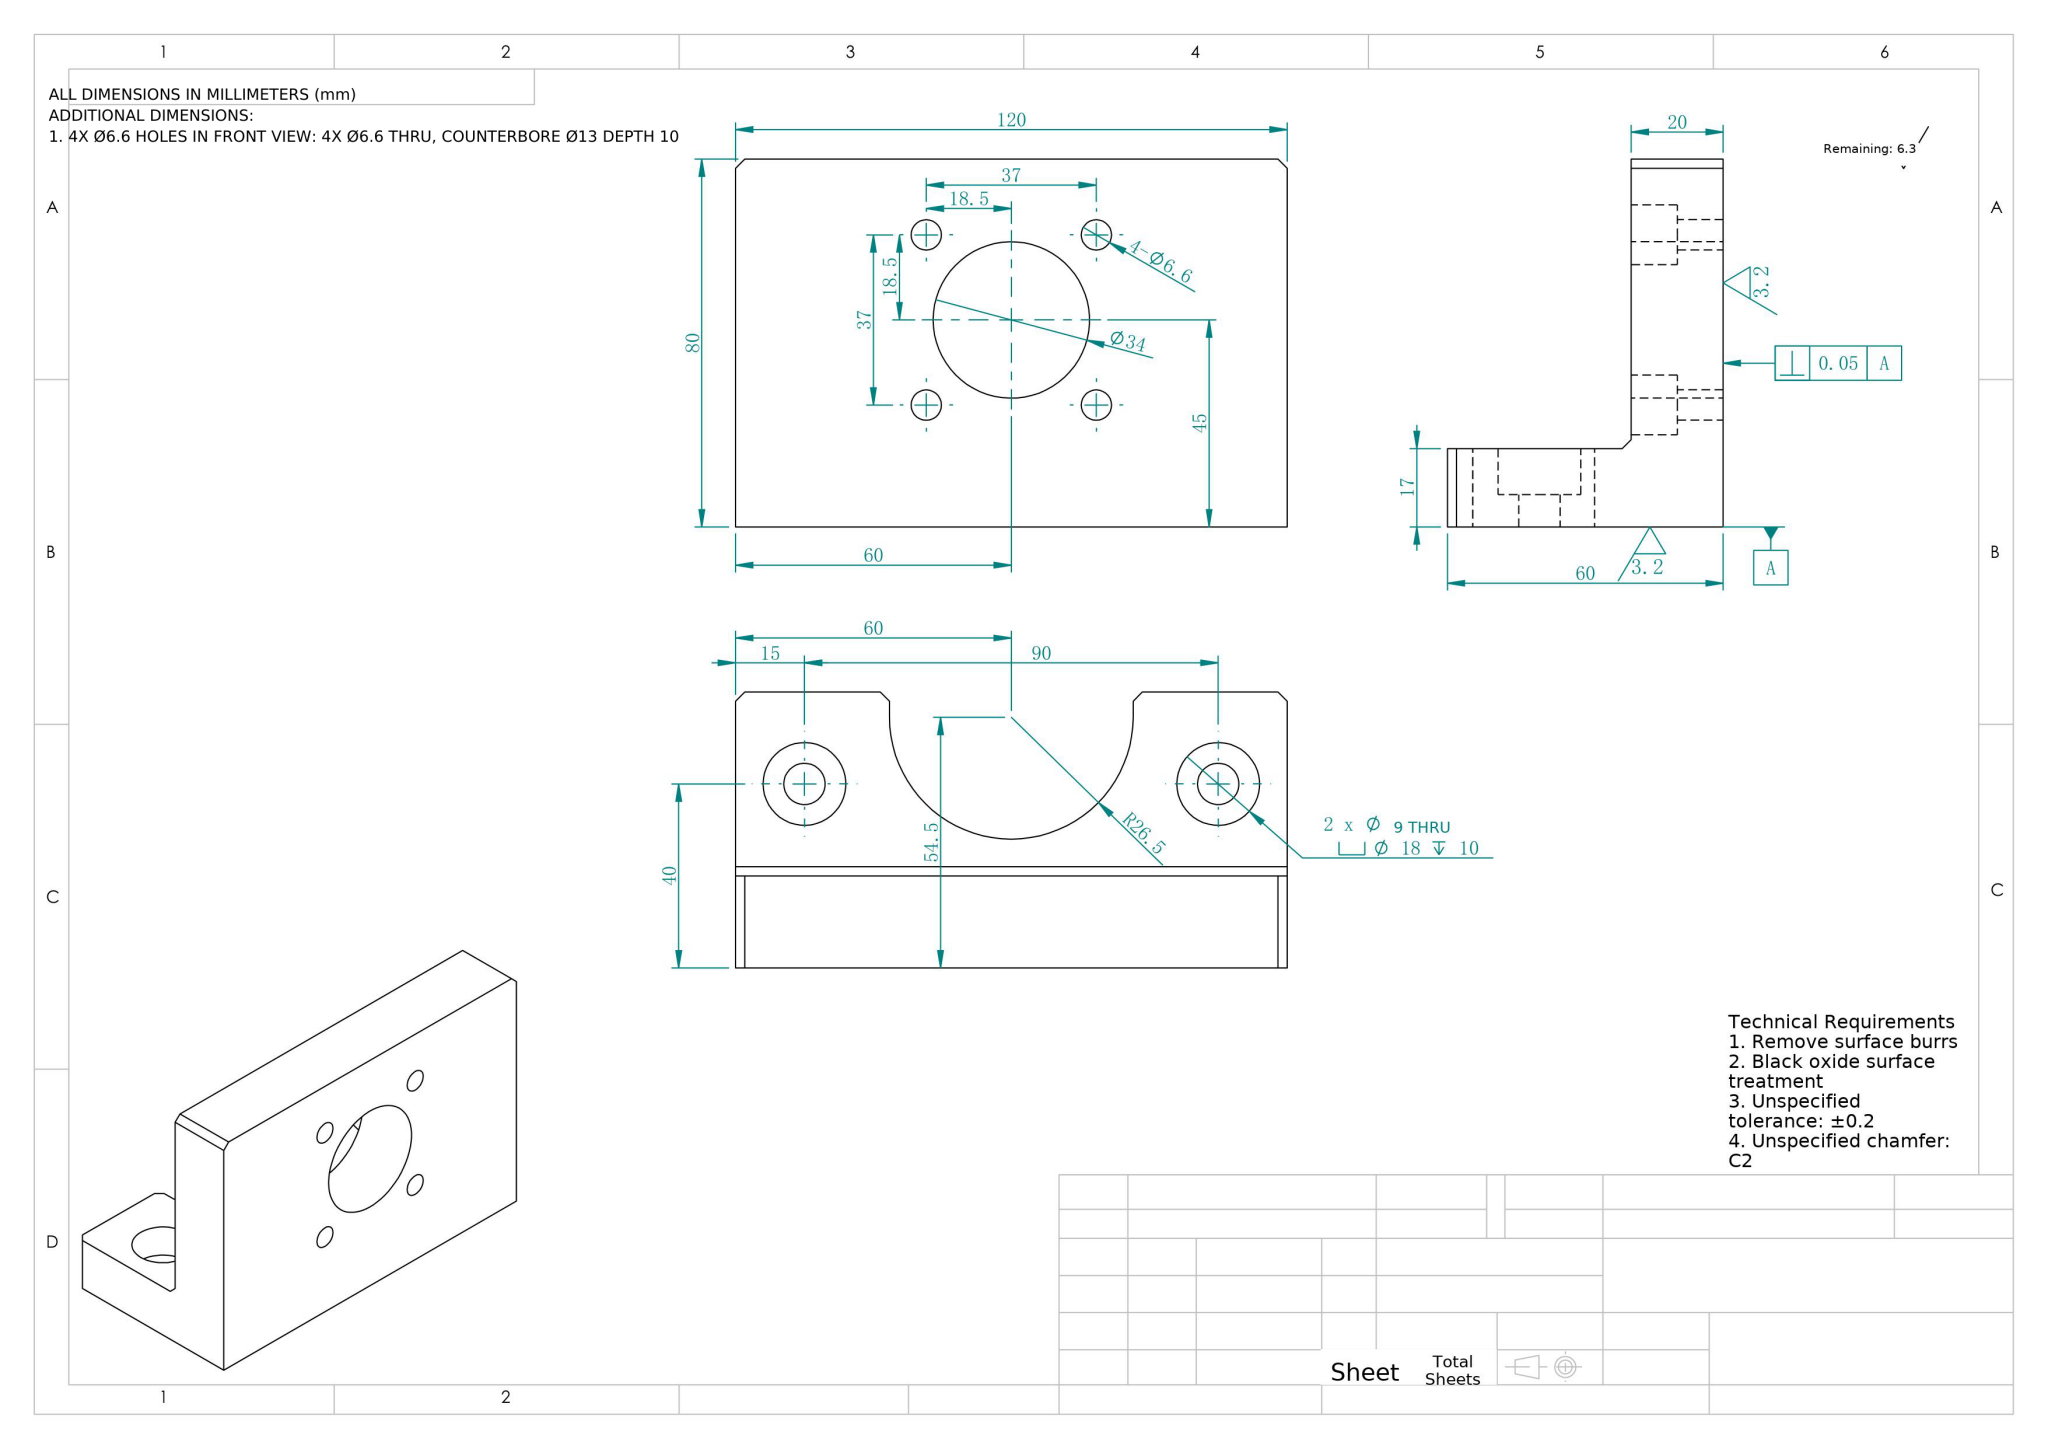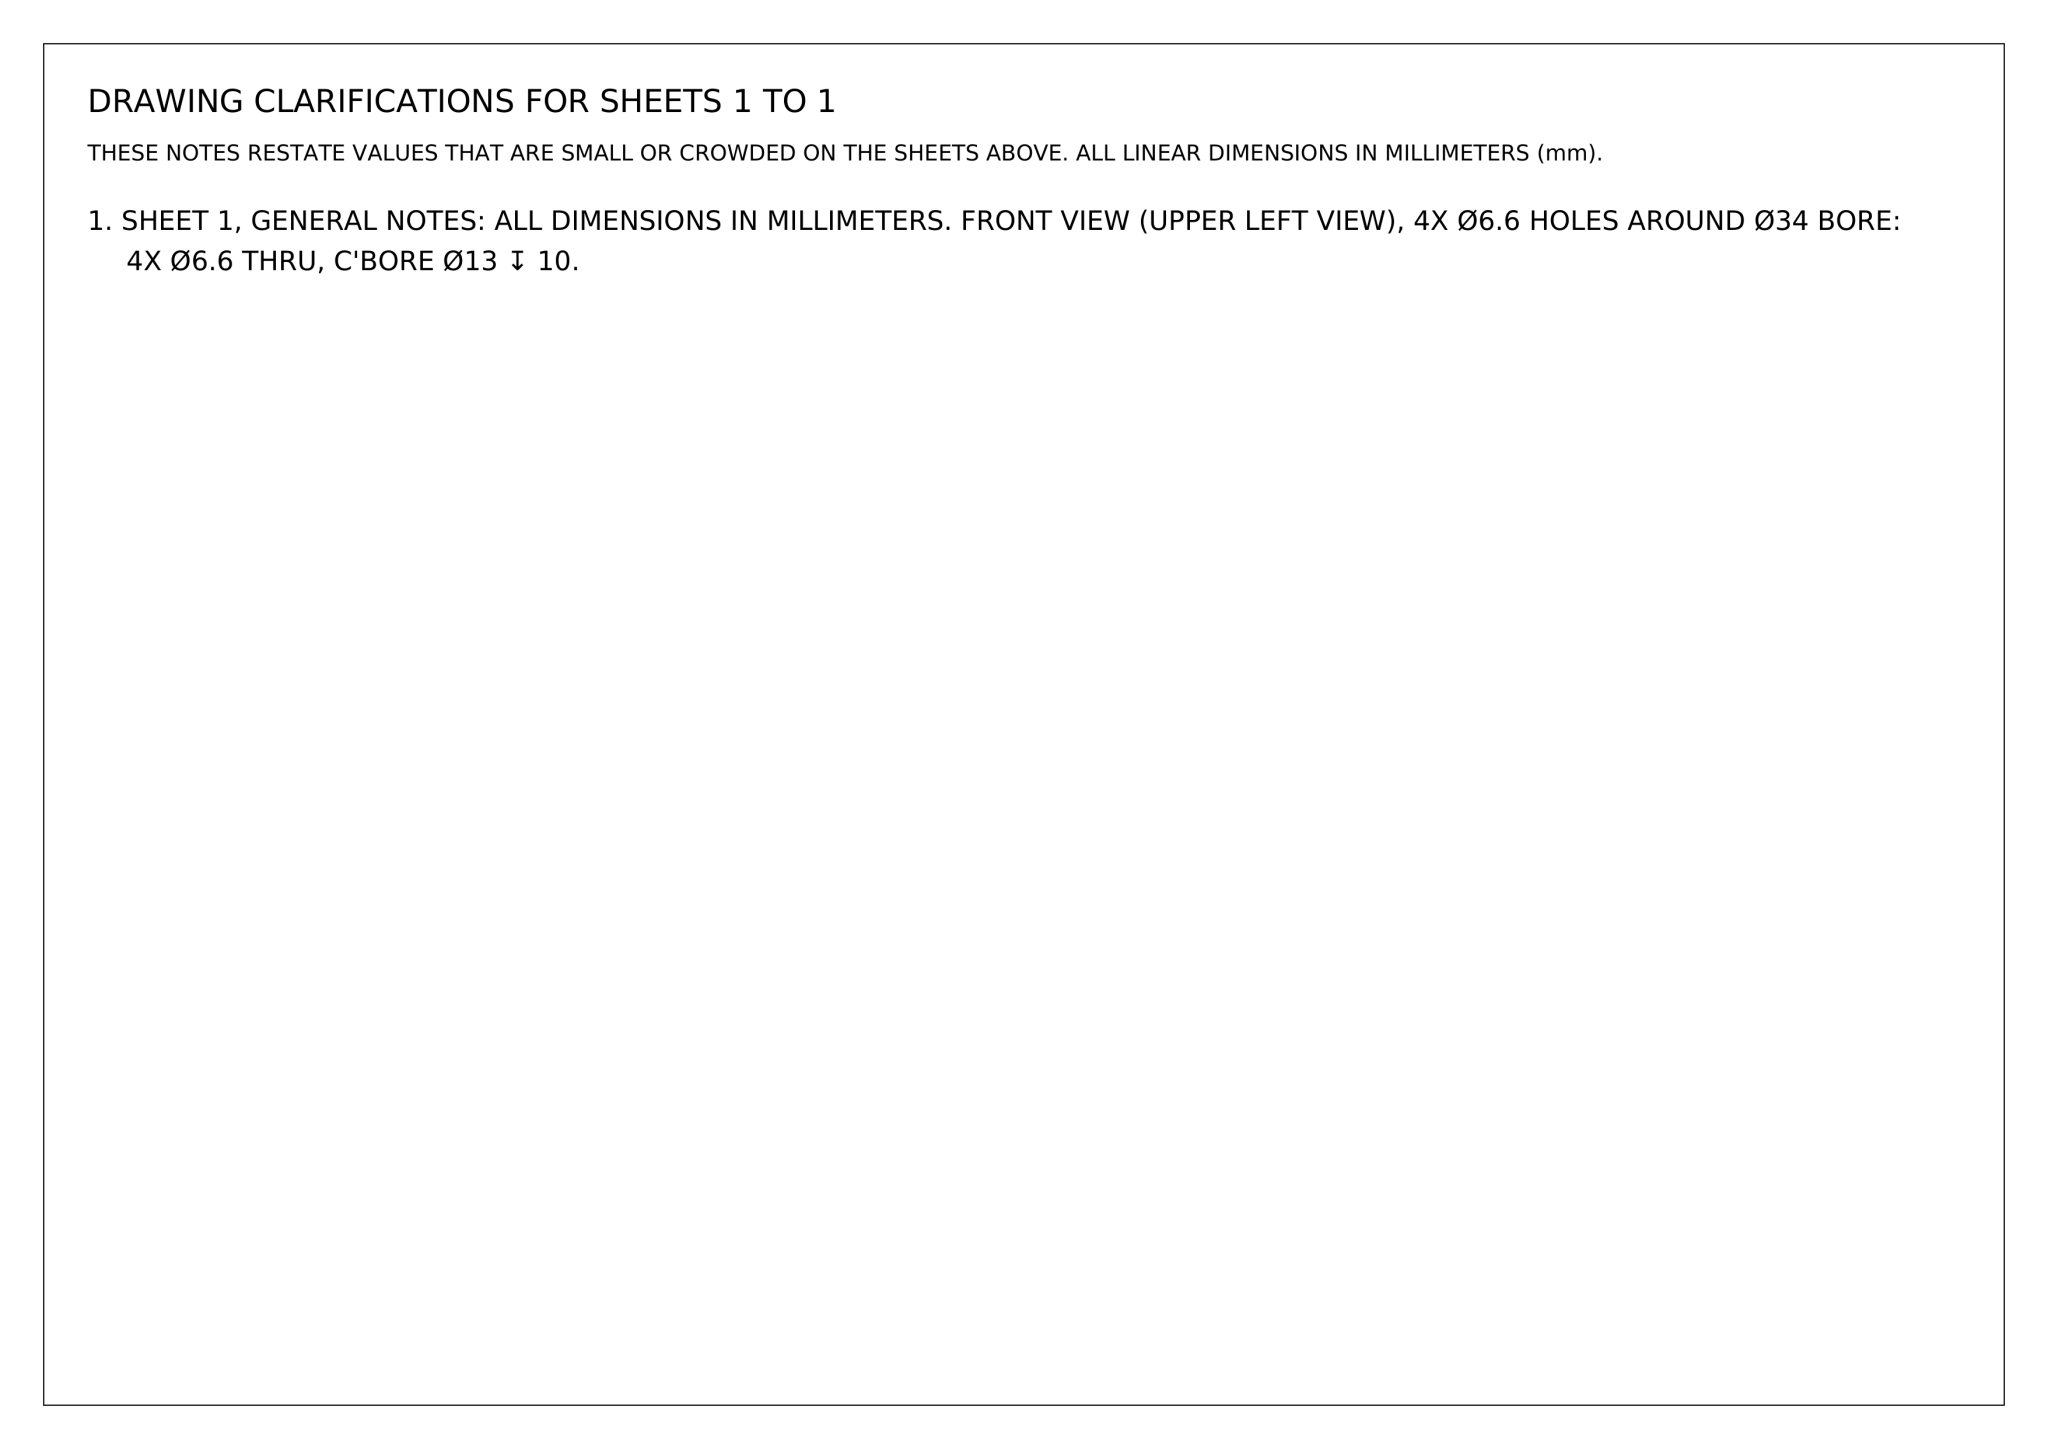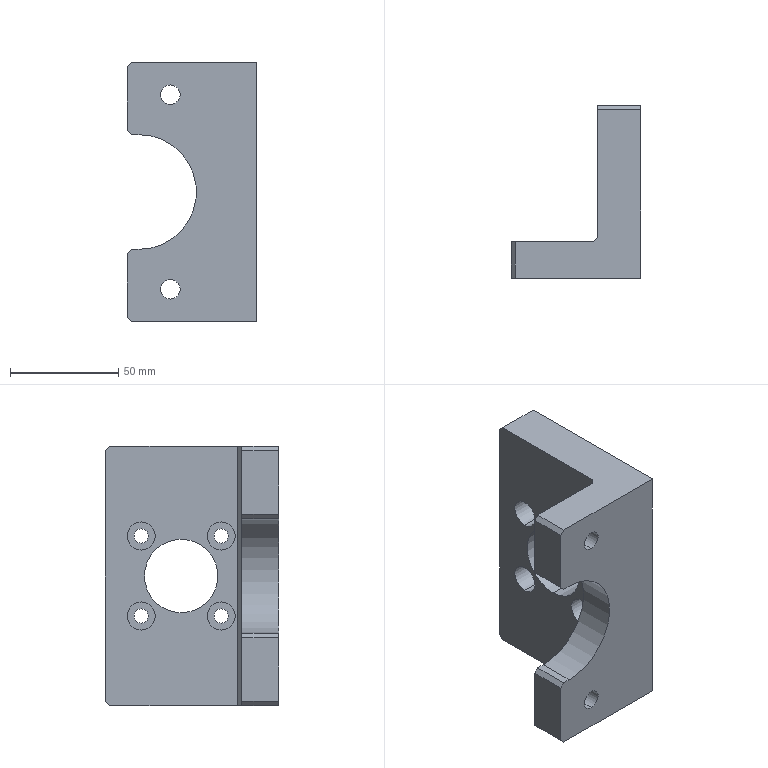Part | NX | mm | 1 solid | 51 faces | box 60 x 80 x 120 mm | volume 219100 mm3 | cylinder 27 | plane 24 | commonest cylinder face diameters 13 x8 6.6 x8 18 x4 9 x4 34 x2 53 x1